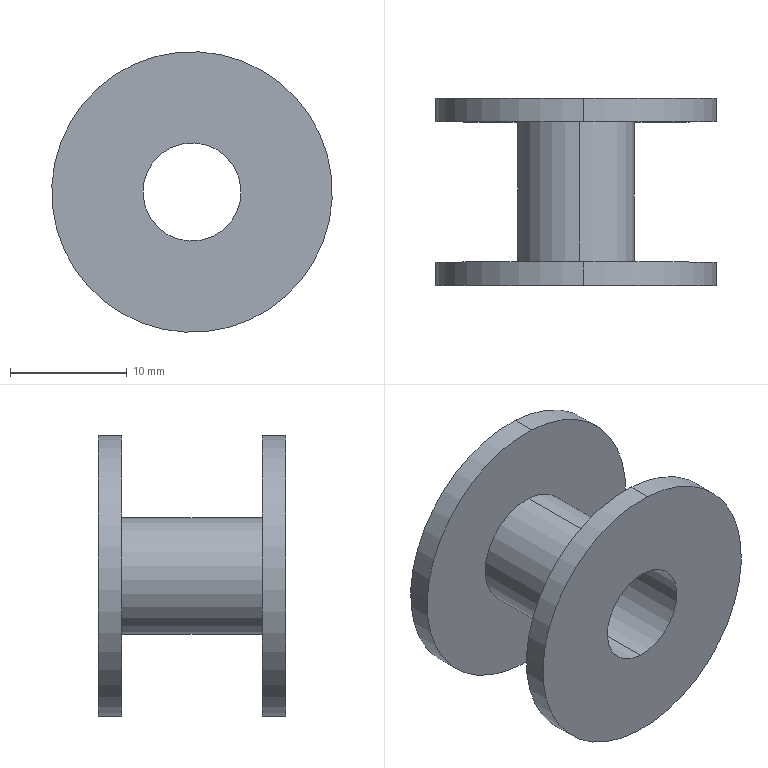Component | SolidWorks | AdhesiveTapeRoll-1 | 1 solid | 12 faces | box 24 x 16 x 24 mm | volume 1865 mm3 | cylinder 8 | plane 4 | commonest cylinder face diameters 24 x4 8.4 x2 10 x2
build123d program:
from build123d import *

# Parameters (mm, degrees)
SKETCH2_R          = 4.2
CUT_EXTRUDE1_DEPTH = 24.324


with BuildPart() as part:
    # Sketch1 → Revolve1 (revolve)
    with BuildSketch(Plane.XY, mode=Mode.PRIVATE) as revolve1_sk:
        Polygon((0, 8.708), (12, 8.708), (12, 6.708), (5, 6.708), (5, -5.292), (12, -5.292), (12, -7.292), (0, -7.292), align=None)
    revolve(revolve1_sk.sketch.rotate(Axis((0, 15.767, 0), (0, -1, 0)), 90), axis=Axis((0, 15.767, 0), (0, -1, 0)))

    # Sketch2 → Cut-Extrude1 (cut, through all)
    with BuildSketch(Plane(origin=(0, 8.708, 0), x_dir=(1, 0, 0), z_dir=(0, 1, 0))):
        with Locations(Location((0, 0, 0), (0, 0, 270))):
            Circle(SKETCH2_R)
    extrude(amount=-CUT_EXTRUDE1_DEPTH, mode=Mode.SUBTRACT)


solid = part.part

# Placed as in the assembly
solid = solid.moved(Location((29.475, -61.208, 229.781), (0, 0, 0)))
STEP:
#1=CARTESIAN_POINT('',(1.152,-2.697,8.881));
#2=VERTEX_POINT('',#1);
#3=CARTESIAN_POINT('',(1.169,-2.697,9.212));
#4=VERTEX_POINT('',#3);
#5=CARTESIAN_POINT('',(1.16,-2.697,9.046));
#6=DIRECTION('',(-0.,1.,-0.));
#7=DIRECTION('',(0.05399,0.,0.9985));
#8=AXIS2_PLACEMENT_3D('',#5,#6,#7);
#9=CIRCLE('',#8,0.1654);
#10=EDGE_CURVE('',#2,#4,#9,.T.);
#11=ORIENTED_EDGE('',*,*,#10,.F.);
#12=CARTESIAN_POINT('',(1.152,-2.067,8.881));
#13=VERTEX_POINT('',#12);
#14=CARTESIAN_POINT('',(1.152,-2.697,8.881));
#15=DIRECTION('',(-0.,1.,-0.));
#16=VECTOR('',#15,39.37);
#17=LINE('',#14,#16);
#18=EDGE_CURVE('',#2,#13,#17,.T.);
#19=ORIENTED_EDGE('',*,*,#18,.T.);
#20=CARTESIAN_POINT('',(1.169,-2.067,9.212));
#21=VERTEX_POINT('',#20);
#22=CARTESIAN_POINT('',(1.16,-2.067,9.046));
#23=DIRECTION('',(-0.,1.,-0.));
#24=DIRECTION('',(0.05399,0.,0.9985));
#25=AXIS2_PLACEMENT_3D('',#22,#23,#24);
#26=CIRCLE('',#25,0.1654);
#27=EDGE_CURVE('',#13,#21,#26,.T.);
#28=ORIENTED_EDGE('',*,*,#27,.T.);
#29=CARTESIAN_POINT('',(1.169,-2.697,9.212));
#30=DIRECTION('',(-0.,1.,-0.));
#31=VECTOR('',#30,39.37);
#32=LINE('',#29,#31);
#33=EDGE_CURVE('',#4,#21,#32,.T.);
#34=ORIENTED_EDGE('',*,*,#33,.F.);
#35=EDGE_LOOP('',(#11,#19,#28,#34));
#36=FACE_OUTER_BOUND('',#35,.T.);
#37=CARTESIAN_POINT('',(1.16,-2.697,9.046));
#38=DIRECTION('',(-0.,1.,-0.));
#39=DIRECTION('',(0.05399,0.,0.9985));
#40=AXIS2_PLACEMENT_3D('',#37,#38,#39);
#41=CYLINDRICAL_SURFACE('',#40,0.1654);
#42=ADVANCED_FACE('',(#36),#41,.F.);
#43=CARTESIAN_POINT('',(1.186,-2.697,9.518));
#44=VERTEX_POINT('',#43);
#45=CARTESIAN_POINT('',(1.135,-2.697,8.575));
#46=VERTEX_POINT('',#45);
#47=CARTESIAN_POINT('',(1.16,-2.697,9.046));
#48=DIRECTION('',(-0.,1.,-0.));
#49=DIRECTION('',(0.05399,0.,0.9985));
#50=AXIS2_PLACEMENT_3D('',#47,#48,#49);
#51=CIRCLE('',#50,0.4724);
#52=EDGE_CURVE('',#44,#46,#51,.T.);
#53=ORIENTED_EDGE('',*,*,#52,.T.);
#54=CARTESIAN_POINT('',(1.135,-2.618,8.575));
#55=VERTEX_POINT('',#54);
#56=CARTESIAN_POINT('',(1.135,-1.789,8.575));
#57=DIRECTION('',(-0.,1.,-0.));
#58=VECTOR('',#57,39.37);
#59=LINE('',#56,#58);
#60=EDGE_CURVE('',#46,#55,#59,.T.);
#61=ORIENTED_EDGE('',*,*,#60,.T.);
#62=CARTESIAN_POINT('',(1.186,-2.618,9.518));
#63=VERTEX_POINT('',#62);
#64=CARTESIAN_POINT('',(1.16,-2.618,9.046));
#65=DIRECTION('',(-0.,1.,-0.));
#66=DIRECTION('',(0.05399,0.,0.9985));
#67=AXIS2_PLACEMENT_3D('',#64,#65,#66);
#68=CIRCLE('',#67,0.4724);
#69=EDGE_CURVE('',#63,#55,#68,.T.);
#70=ORIENTED_EDGE('',*,*,#69,.F.);
#71=CARTESIAN_POINT('',(1.186,-1.789,9.518));
#72=DIRECTION('',(-0.,1.,-0.));
#73=VECTOR('',#72,39.37);
#74=LINE('',#71,#73);
#75=EDGE_CURVE('',#44,#63,#74,.T.);
#76=ORIENTED_EDGE('',*,*,#75,.F.);
#77=EDGE_LOOP('',(#53,#61,#70,#76));
#78=FACE_OUTER_BOUND('',#77,.T.);
#79=CARTESIAN_POINT('',(1.16,-1.789,9.046));
#80=DIRECTION('',(-0.,1.,-0.));
#81=DIRECTION('',(0.05399,0.,0.9985));
#82=AXIS2_PLACEMENT_3D('',#79,#80,#81);
#83=CYLINDRICAL_SURFACE('',#82,0.4724);
#84=ADVANCED_FACE('',(#78),#83,.T.);
#85=CARTESIAN_POINT('',(1.171,-2.618,9.243));
#86=VERTEX_POINT('',#85);
#87=CARTESIAN_POINT('',(1.15,-2.618,8.85));
#88=VERTEX_POINT('',#87);
#89=CARTESIAN_POINT('',(1.16,-2.618,9.046));
#90=DIRECTION('',(-0.,1.,-0.));
#91=DIRECTION('',(0.05399,0.,0.9985));
#92=AXIS2_PLACEMENT_3D('',#89,#90,#91);
#93=CIRCLE('',#92,0.1969);
#94=EDGE_CURVE('',#86,#88,#93,.T.);
#95=ORIENTED_EDGE('',*,*,#94,.T.);
#96=CARTESIAN_POINT('',(1.15,-2.146,8.85));
#97=VERTEX_POINT('',#96);
#98=CARTESIAN_POINT('',(1.15,-1.789,8.85));
#99=DIRECTION('',(-0.,1.,-0.));
#100=VECTOR('',#99,39.37);
#101=LINE('',#98,#100);
#102=EDGE_CURVE('',#88,#97,#101,.T.);
#103=ORIENTED_EDGE('',*,*,#102,.T.);
#104=CARTESIAN_POINT('',(1.171,-2.146,9.243));
#105=VERTEX_POINT('',#104);
#106=CARTESIAN_POINT('',(1.16,-2.146,9.046));
#107=DIRECTION('',(-0.,1.,-0.));
#108=DIRECTION('',(0.05399,0.,0.9985));
#109=AXIS2_PLACEMENT_3D('',#106,#107,#108);
#110=CIRCLE('',#109,0.1969);
#111=EDGE_CURVE('',#105,#97,#110,.T.);
#112=ORIENTED_EDGE('',*,*,#111,.F.);
#113=CARTESIAN_POINT('',(1.171,-1.789,9.243));
#114=DIRECTION('',(-0.,1.,-0.));
#115=VECTOR('',#114,39.37);
#116=LINE('',#113,#115);
#117=EDGE_CURVE('',#86,#105,#116,.T.);
#118=ORIENTED_EDGE('',*,*,#117,.F.);
#119=EDGE_LOOP('',(#95,#103,#112,#118));
#120=FACE_OUTER_BOUND('',#119,.T.);
#121=CARTESIAN_POINT('',(1.16,-1.789,9.046));
#122=DIRECTION('',(-0.,1.,-0.));
#123=DIRECTION('',(0.05399,0.,0.9985));
#124=AXIS2_PLACEMENT_3D('',#121,#122,#123);
#125=CYLINDRICAL_SURFACE('',#124,0.1969);
#126=ADVANCED_FACE('',(#120),#125,.T.);
#127=CARTESIAN_POINT('',(1.186,-2.146,9.518));
#128=VERTEX_POINT('',#127);
#129=CARTESIAN_POINT('',(1.135,-2.146,8.575));
#130=VERTEX_POINT('',#129);
#131=CARTESIAN_POINT('',(1.16,-2.146,9.046));
#132=DIRECTION('',(-0.,1.,-0.));
#133=DIRECTION('',(0.05399,0.,0.9985));
#134=AXIS2_PLACEMENT_3D('',#131,#132,#133);
#135=CIRCLE('',#134,0.4724);
#136=EDGE_CURVE('',#128,#130,#135,.T.);
#137=ORIENTED_EDGE('',*,*,#136,.T.);
#138=CARTESIAN_POINT('',(1.135,-2.067,8.575));
#139=VERTEX_POINT('',#138);
#140=CARTESIAN_POINT('',(1.135,-1.789,8.575));
#141=DIRECTION('',(-0.,1.,-0.));
#142=VECTOR('',#141,39.37);
#143=LINE('',#140,#142);
#144=EDGE_CURVE('',#130,#139,#143,.T.);
#145=ORIENTED_EDGE('',*,*,#144,.T.);
#146=CARTESIAN_POINT('',(1.186,-2.067,9.518));
#147=VERTEX_POINT('',#146);
#148=CARTESIAN_POINT('',(1.16,-2.067,9.046));
#149=DIRECTION('',(-0.,1.,-0.));
#150=DIRECTION('',(0.05399,0.,0.9985));
#151=AXIS2_PLACEMENT_3D('',#148,#149,#150);
#152=CIRCLE('',#151,0.4724);
#153=EDGE_CURVE('',#147,#139,#152,.T.);
#154=ORIENTED_EDGE('',*,*,#153,.F.);
#155=CARTESIAN_POINT('',(1.186,-1.789,9.518));
#156=DIRECTION('',(-0.,1.,-0.));
#157=VECTOR('',#156,39.37);
#158=LINE('',#155,#157);
#159=EDGE_CURVE('',#128,#147,#158,.T.);
#160=ORIENTED_EDGE('',*,*,#159,.F.);
#161=EDGE_LOOP('',(#137,#145,#154,#160));
#162=FACE_OUTER_BOUND('',#161,.T.);
#163=CARTESIAN_POINT('',(1.16,-1.789,9.046));
#164=DIRECTION('',(-0.,1.,-0.));
#165=DIRECTION('',(0.05399,0.,0.9985));
#166=AXIS2_PLACEMENT_3D('',#163,#164,#165);
#167=CYLINDRICAL_SURFACE('',#166,0.4724);
#168=ADVANCED_FACE('',(#162),#167,.T.);
#169=CARTESIAN_POINT('',(1.16,-2.067,9.046));
#170=DIRECTION('',(-0.,1.,-0.));
#171=DIRECTION('',(0.05399,0.,0.9985));
#172=AXIS2_PLACEMENT_3D('',#169,#170,#171);
#173=CIRCLE('',#172,0.1654);
#174=EDGE_CURVE('',#21,#13,#173,.T.);
#175=ORIENTED_EDGE('',*,*,#174,.F.);
#176=ORIENTED_EDGE('',*,*,#27,.F.);
#177=EDGE_LOOP('',(#175,#176));
#178=FACE_BOUND('',#177,.T.);
#179=ORIENTED_EDGE('',*,*,#153,.T.);
#180=CARTESIAN_POINT('',(1.16,-2.067,9.046));
#181=DIRECTION('',(-0.,1.,-0.));
#182=DIRECTION('',(0.05399,0.,0.9985));
#183=AXIS2_PLACEMENT_3D('',#180,#181,#182);
#184=CIRCLE('',#183,0.4724);
#185=EDGE_CURVE('',#139,#147,#184,.T.);
#186=ORIENTED_EDGE('',*,*,#185,.T.);
#187=EDGE_LOOP('',(#179,#186));
#188=FACE_OUTER_BOUND('',#187,.T.);
#189=CARTESIAN_POINT('',(1.16,-2.067,9.046));
#190=DIRECTION('',(0.,-1.,0.));
#191=DIRECTION('',(-0.05399,-0.,-0.9985));
#192=AXIS2_PLACEMENT_3D('',#189,#190,#191);
#193=PLANE('',#192);
#194=ADVANCED_FACE('',(#178,#188),#193,.F.);
#195=ORIENTED_EDGE('',*,*,#144,.F.);
#196=CARTESIAN_POINT('',(1.16,-2.146,9.046));
#197=DIRECTION('',(-0.,1.,-0.));
#198=DIRECTION('',(0.05399,0.,0.9985));
#199=AXIS2_PLACEMENT_3D('',#196,#197,#198);
#200=CIRCLE('',#199,0.4724);
#201=EDGE_CURVE('',#130,#128,#200,.T.);
#202=ORIENTED_EDGE('',*,*,#201,.T.);
#203=ORIENTED_EDGE('',*,*,#159,.T.);
#204=ORIENTED_EDGE('',*,*,#185,.F.);
#205=EDGE_LOOP('',(#195,#202,#203,#204));
#206=FACE_OUTER_BOUND('',#205,.T.);
#207=CARTESIAN_POINT('',(1.16,-1.789,9.046));
#208=DIRECTION('',(-0.,1.,-0.));
#209=DIRECTION('',(0.05399,0.,0.9985));
#210=AXIS2_PLACEMENT_3D('',#207,#208,#209);
#211=CYLINDRICAL_SURFACE('',#210,0.4724);
#212=ADVANCED_FACE('',(#206),#211,.T.);
#213=ORIENTED_EDGE('',*,*,#136,.F.);
#214=ORIENTED_EDGE('',*,*,#201,.F.);
#215=EDGE_LOOP('',(#213,#214));
#216=FACE_OUTER_BOUND('',#215,.T.);
#217=ORIENTED_EDGE('',*,*,#111,.T.);
#218=CARTESIAN_POINT('',(1.16,-2.146,9.046));
#219=DIRECTION('',(-0.,1.,-0.));
#220=DIRECTION('',(0.05399,0.,0.9985));
#221=AXIS2_PLACEMENT_3D('',#218,#219,#220);
#222=CIRCLE('',#221,0.1969);
#223=EDGE_CURVE('',#97,#105,#222,.T.);
#224=ORIENTED_EDGE('',*,*,#223,.T.);
#225=EDGE_LOOP('',(#217,#224));
#226=FACE_BOUND('',#225,.T.);
#227=CARTESIAN_POINT('',(1.632,-2.146,9.021));
#228=DIRECTION('',(-0.,1.,-0.));
#229=DIRECTION('',(0.05399,0.,0.9985));
#230=AXIS2_PLACEMENT_3D('',#227,#228,#229);
#231=PLANE('',#230);
#232=ADVANCED_FACE('',(#216,#226),#231,.F.);
#233=ORIENTED_EDGE('',*,*,#102,.F.);
#234=CARTESIAN_POINT('',(1.16,-2.618,9.046));
#235=DIRECTION('',(-0.,1.,-0.));
#236=DIRECTION('',(0.05399,0.,0.9985));
#237=AXIS2_PLACEMENT_3D('',#234,#235,#236);
#238=CIRCLE('',#237,0.1969);
#239=EDGE_CURVE('',#88,#86,#238,.T.);
#240=ORIENTED_EDGE('',*,*,#239,.T.);
#241=ORIENTED_EDGE('',*,*,#117,.T.);
#242=ORIENTED_EDGE('',*,*,#223,.F.);
#243=EDGE_LOOP('',(#233,#240,#241,#242));
#244=FACE_OUTER_BOUND('',#243,.T.);
#245=CARTESIAN_POINT('',(1.16,-1.789,9.046));
#246=DIRECTION('',(-0.,1.,-0.));
#247=DIRECTION('',(0.05399,0.,0.9985));
#248=AXIS2_PLACEMENT_3D('',#245,#246,#247);
#249=CYLINDRICAL_SURFACE('',#248,0.1969);
#250=ADVANCED_FACE('',(#244),#249,.T.);
#251=ORIENTED_EDGE('',*,*,#94,.F.);
#252=ORIENTED_EDGE('',*,*,#239,.F.);
#253=EDGE_LOOP('',(#251,#252));
#254=FACE_BOUND('',#253,.T.);
#255=ORIENTED_EDGE('',*,*,#69,.T.);
#256=CARTESIAN_POINT('',(1.16,-2.618,9.046));
#257=DIRECTION('',(-0.,1.,-0.));
#258=DIRECTION('',(0.05399,0.,0.9985));
#259=AXIS2_PLACEMENT_3D('',#256,#257,#258);
#260=CIRCLE('',#259,0.4724);
#261=EDGE_CURVE('',#55,#63,#260,.T.);
#262=ORIENTED_EDGE('',*,*,#261,.T.);
#263=EDGE_LOOP('',(#255,#262));
#264=FACE_OUTER_BOUND('',#263,.T.);
#265=CARTESIAN_POINT('',(1.357,-2.618,9.036));
#266=DIRECTION('',(0.,-1.,0.));
#267=DIRECTION('',(-0.05399,-0.,-0.9985));
#268=AXIS2_PLACEMENT_3D('',#265,#266,#267);
#269=PLANE('',#268);
#270=ADVANCED_FACE('',(#254,#264),#269,.F.);
#271=ORIENTED_EDGE('',*,*,#60,.F.);
#272=CARTESIAN_POINT('',(1.16,-2.697,9.046));
#273=DIRECTION('',(-0.,1.,-0.));
#274=DIRECTION('',(0.05399,0.,0.9985));
#275=AXIS2_PLACEMENT_3D('',#272,#273,#274);
#276=CIRCLE('',#275,0.4724);
#277=EDGE_CURVE('',#46,#44,#276,.T.);
#278=ORIENTED_EDGE('',*,*,#277,.T.);
#279=ORIENTED_EDGE('',*,*,#75,.T.);
#280=ORIENTED_EDGE('',*,*,#261,.F.);
#281=EDGE_LOOP('',(#271,#278,#279,#280));
#282=FACE_OUTER_BOUND('',#281,.T.);
#283=CARTESIAN_POINT('',(1.16,-1.789,9.046));
#284=DIRECTION('',(-0.,1.,-0.));
#285=DIRECTION('',(0.05399,0.,0.9985));
#286=AXIS2_PLACEMENT_3D('',#283,#284,#285);
#287=CYLINDRICAL_SURFACE('',#286,0.4724);
#288=ADVANCED_FACE('',(#282),#287,.T.);
#289=CARTESIAN_POINT('',(1.16,-2.697,9.046));
#290=DIRECTION('',(-0.,1.,-0.));
#291=DIRECTION('',(0.05399,0.,0.9985));
#292=AXIS2_PLACEMENT_3D('',#289,#290,#291);
#293=CIRCLE('',#292,0.1654);
#294=EDGE_CURVE('',#4,#2,#293,.T.);
#295=ORIENTED_EDGE('',*,*,#294,.T.);
#296=ORIENTED_EDGE('',*,*,#10,.T.);
#297=EDGE_LOOP('',(#295,#296));
#298=FACE_BOUND('',#297,.T.);
#299=ORIENTED_EDGE('',*,*,#52,.F.);
#300=ORIENTED_EDGE('',*,*,#277,.F.);
#301=EDGE_LOOP('',(#299,#300));
#302=FACE_OUTER_BOUND('',#301,.T.);
#303=CARTESIAN_POINT('',(1.632,-2.697,9.021));
#304=DIRECTION('',(-0.,1.,-0.));
#305=DIRECTION('',(0.05399,0.,0.9985));
#306=AXIS2_PLACEMENT_3D('',#303,#304,#305);
#307=PLANE('',#306);
#308=ADVANCED_FACE('',(#298,#302),#307,.F.);
#309=ORIENTED_EDGE('',*,*,#18,.F.);
#310=ORIENTED_EDGE('',*,*,#294,.F.);
#311=ORIENTED_EDGE('',*,*,#33,.T.);
#312=ORIENTED_EDGE('',*,*,#174,.T.);
#313=EDGE_LOOP('',(#309,#310,#311,#312));
#314=FACE_OUTER_BOUND('',#313,.T.);
#315=CARTESIAN_POINT('',(1.16,-2.697,9.046));
#316=DIRECTION('',(-0.,1.,-0.));
#317=DIRECTION('',(0.05399,0.,0.9985));
#318=AXIS2_PLACEMENT_3D('',#315,#316,#317);
#319=CYLINDRICAL_SURFACE('',#318,0.1654);
#320=ADVANCED_FACE('',(#314),#319,.F.);
#321=CLOSED_SHELL('',(#42,#84,#126,#168,#194,#212,#232,#250,#270,#288,#308,#320));
#322=MANIFOLD_SOLID_BREP('',#321);
#323=CARTESIAN_POINT('',(0.,0.,0.));
#324=DIRECTION('',(0.,0.,1.));
#325=DIRECTION('',(1.,0.,0.));
#326=AXIS2_PLACEMENT_3D('',#323,#324,#325);
#327=(LENGTH_UNIT()NAMED_UNIT(*)SI_UNIT($,.METRE.));
#328=LENGTH_MEASURE_WITH_UNIT(LENGTH_MEASURE(0.0254),#327);
#329=DIMENSIONAL_EXPONENTS(1.,0.,0.,0.,0.,0.,0.);
#330=(CONVERSION_BASED_UNIT('',#328)LENGTH_UNIT()NAMED_UNIT(#329));
#331=UNCERTAINTY_MEASURE_WITH_UNIT(LENGTH_MEASURE(0.00001),#330,'','');
#332=(NAMED_UNIT(*)PLANE_ANGLE_UNIT()SI_UNIT($,.RADIAN.));
#333=(NAMED_UNIT(*)SI_UNIT($,.STERADIAN.)SOLID_ANGLE_UNIT());
#334=(GEOMETRIC_REPRESENTATION_CONTEXT(3)GLOBAL_UNCERTAINTY_ASSIGNED_CONTEXT((#331))GLOBAL_UNIT_ASSIGNED_CONTEXT((#330,#332,#333))REPRESENTATION_CONTEXT('',''));
#335=ADVANCED_BREP_SHAPE_REPRESENTATION('',(#322,#326),#334);
#336=COLOUR_RGB('',0.7922,0.8196,0.9333);
#337=FILL_AREA_STYLE_COLOUR('',#336);
#338=FILL_AREA_STYLE('',(#337));
#339=SURFACE_STYLE_FILL_AREA(#338);
#340=SURFACE_SIDE_STYLE('',(#339));
#341=SURFACE_STYLE_USAGE(.BOTH.,#340);
#342=PRESENTATION_STYLE_ASSIGNMENT((#341));
#343=STYLED_ITEM('',(#342),#322);
#344=PRESENTATION_LAYER_ASSIGNMENT('','',(#343));
#345=(LENGTH_UNIT()NAMED_UNIT(*)SI_UNIT($,.METRE.));
#346=LENGTH_MEASURE_WITH_UNIT(LENGTH_MEASURE(0.0254),#345);
#347=DIMENSIONAL_EXPONENTS(1.,0.,0.,0.,0.,0.,0.);
#348=(CONVERSION_BASED_UNIT('',#346)LENGTH_UNIT()NAMED_UNIT(#347));
#349=UNCERTAINTY_MEASURE_WITH_UNIT(LENGTH_MEASURE(0.00001),#348,'','');
#350=(NAMED_UNIT(*)PLANE_ANGLE_UNIT()SI_UNIT($,.RADIAN.));
#351=(NAMED_UNIT(*)SI_UNIT($,.STERADIAN.)SOLID_ANGLE_UNIT());
#352=(GEOMETRIC_REPRESENTATION_CONTEXT(3)GLOBAL_UNCERTAINTY_ASSIGNED_CONTEXT((#349))GLOBAL_UNIT_ASSIGNED_CONTEXT((#348,#350,#351))REPRESENTATION_CONTEXT('',''));
#353=MECHANICAL_DESIGN_GEOMETRIC_PRESENTATION_REPRESENTATION('',(#343),#352);